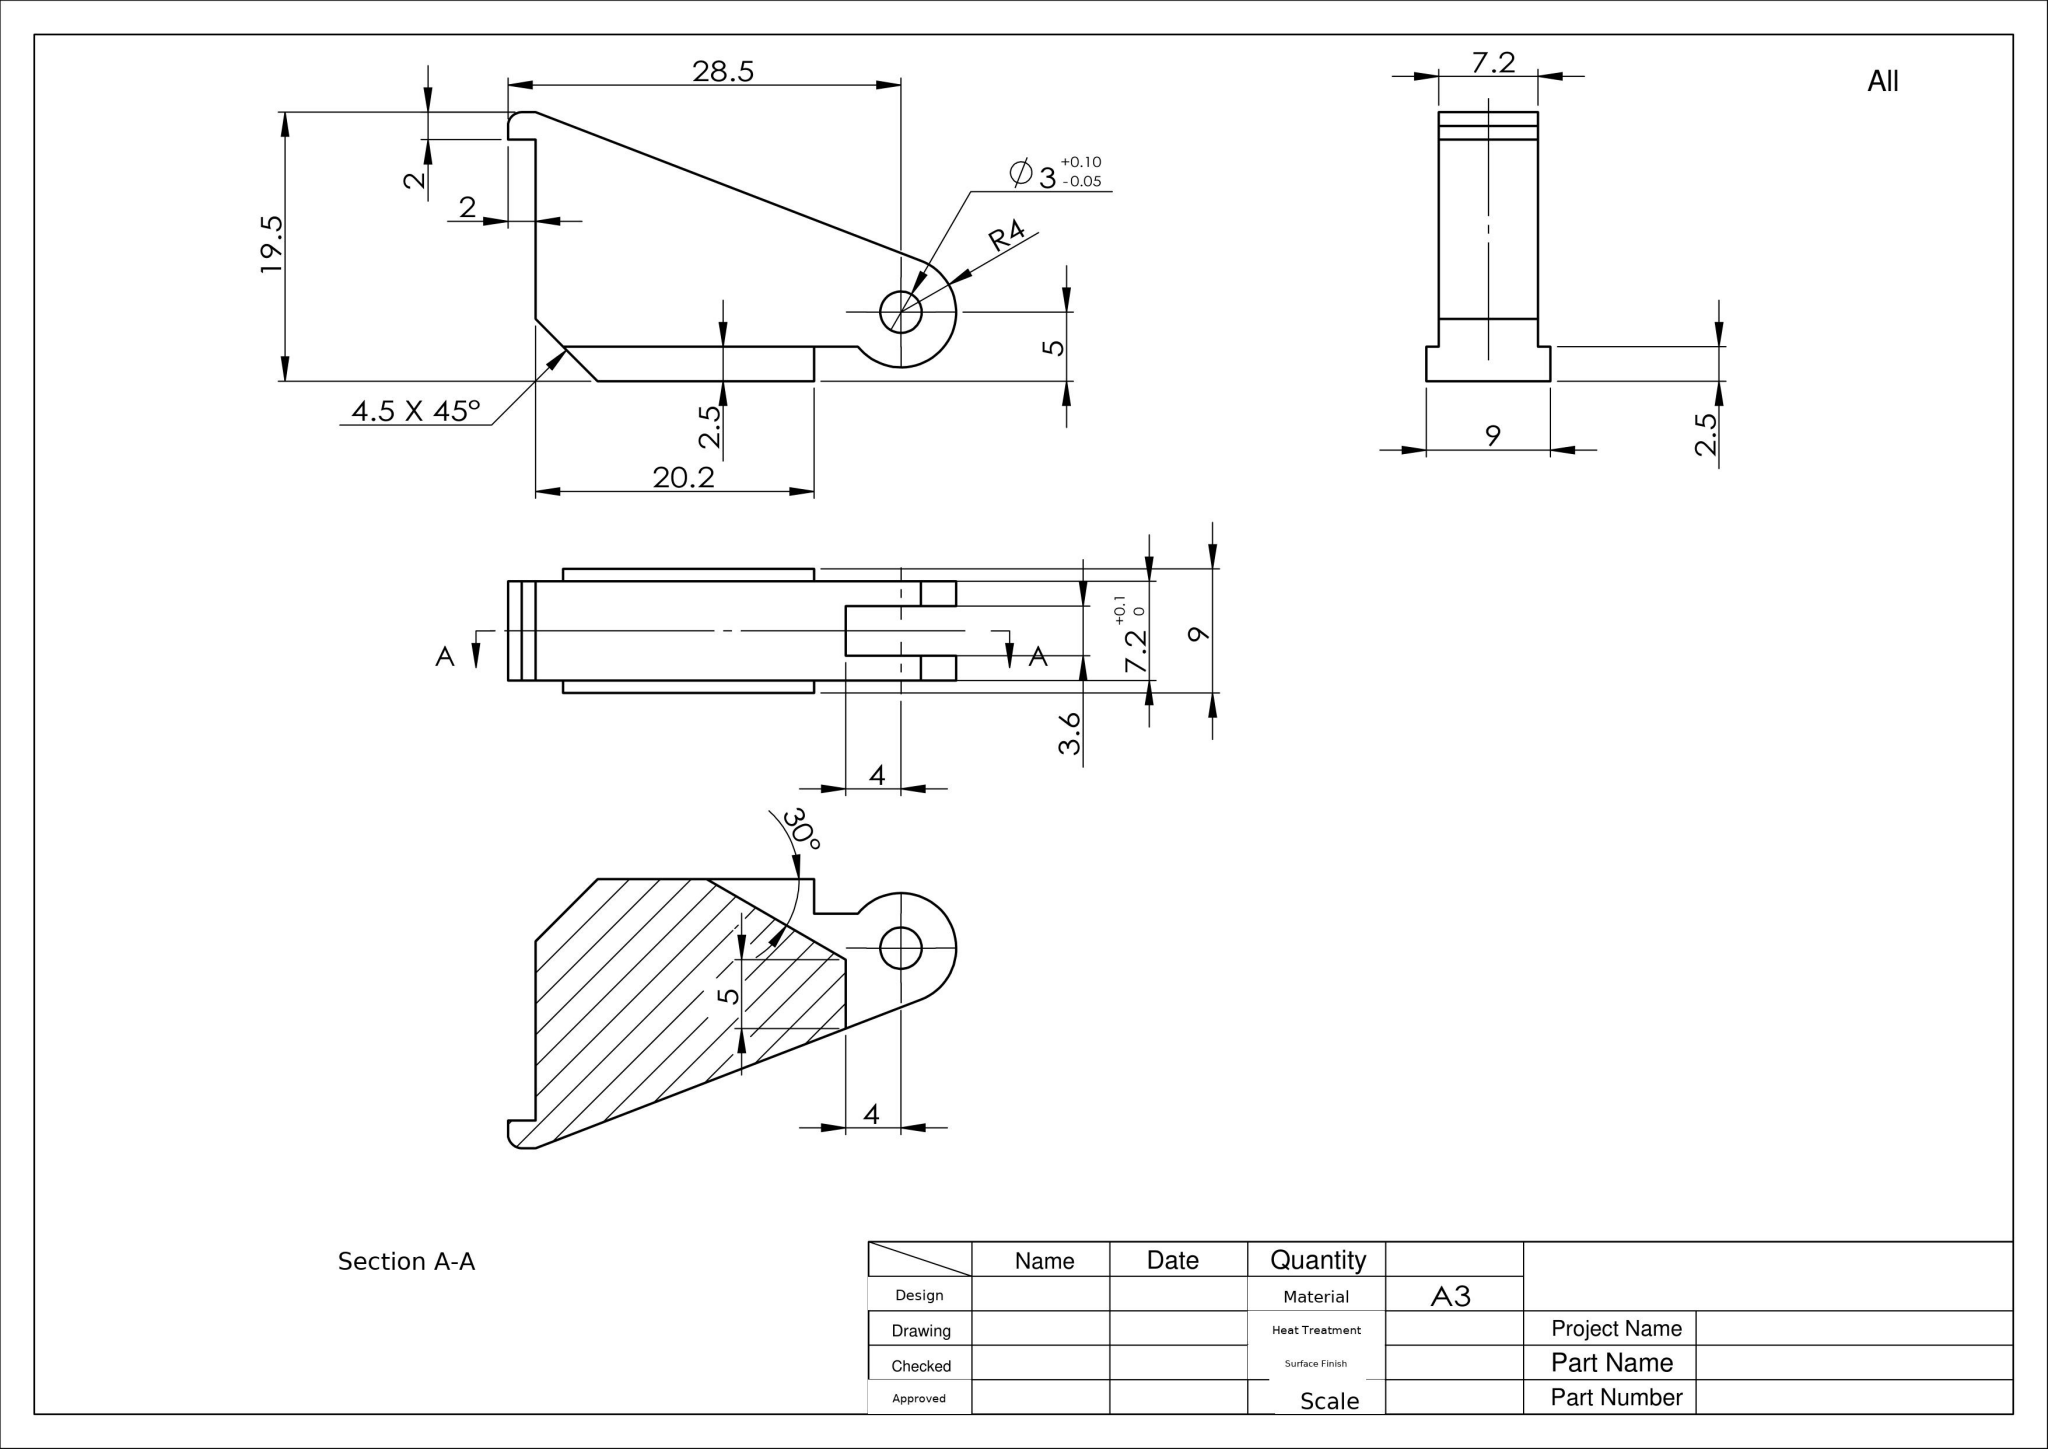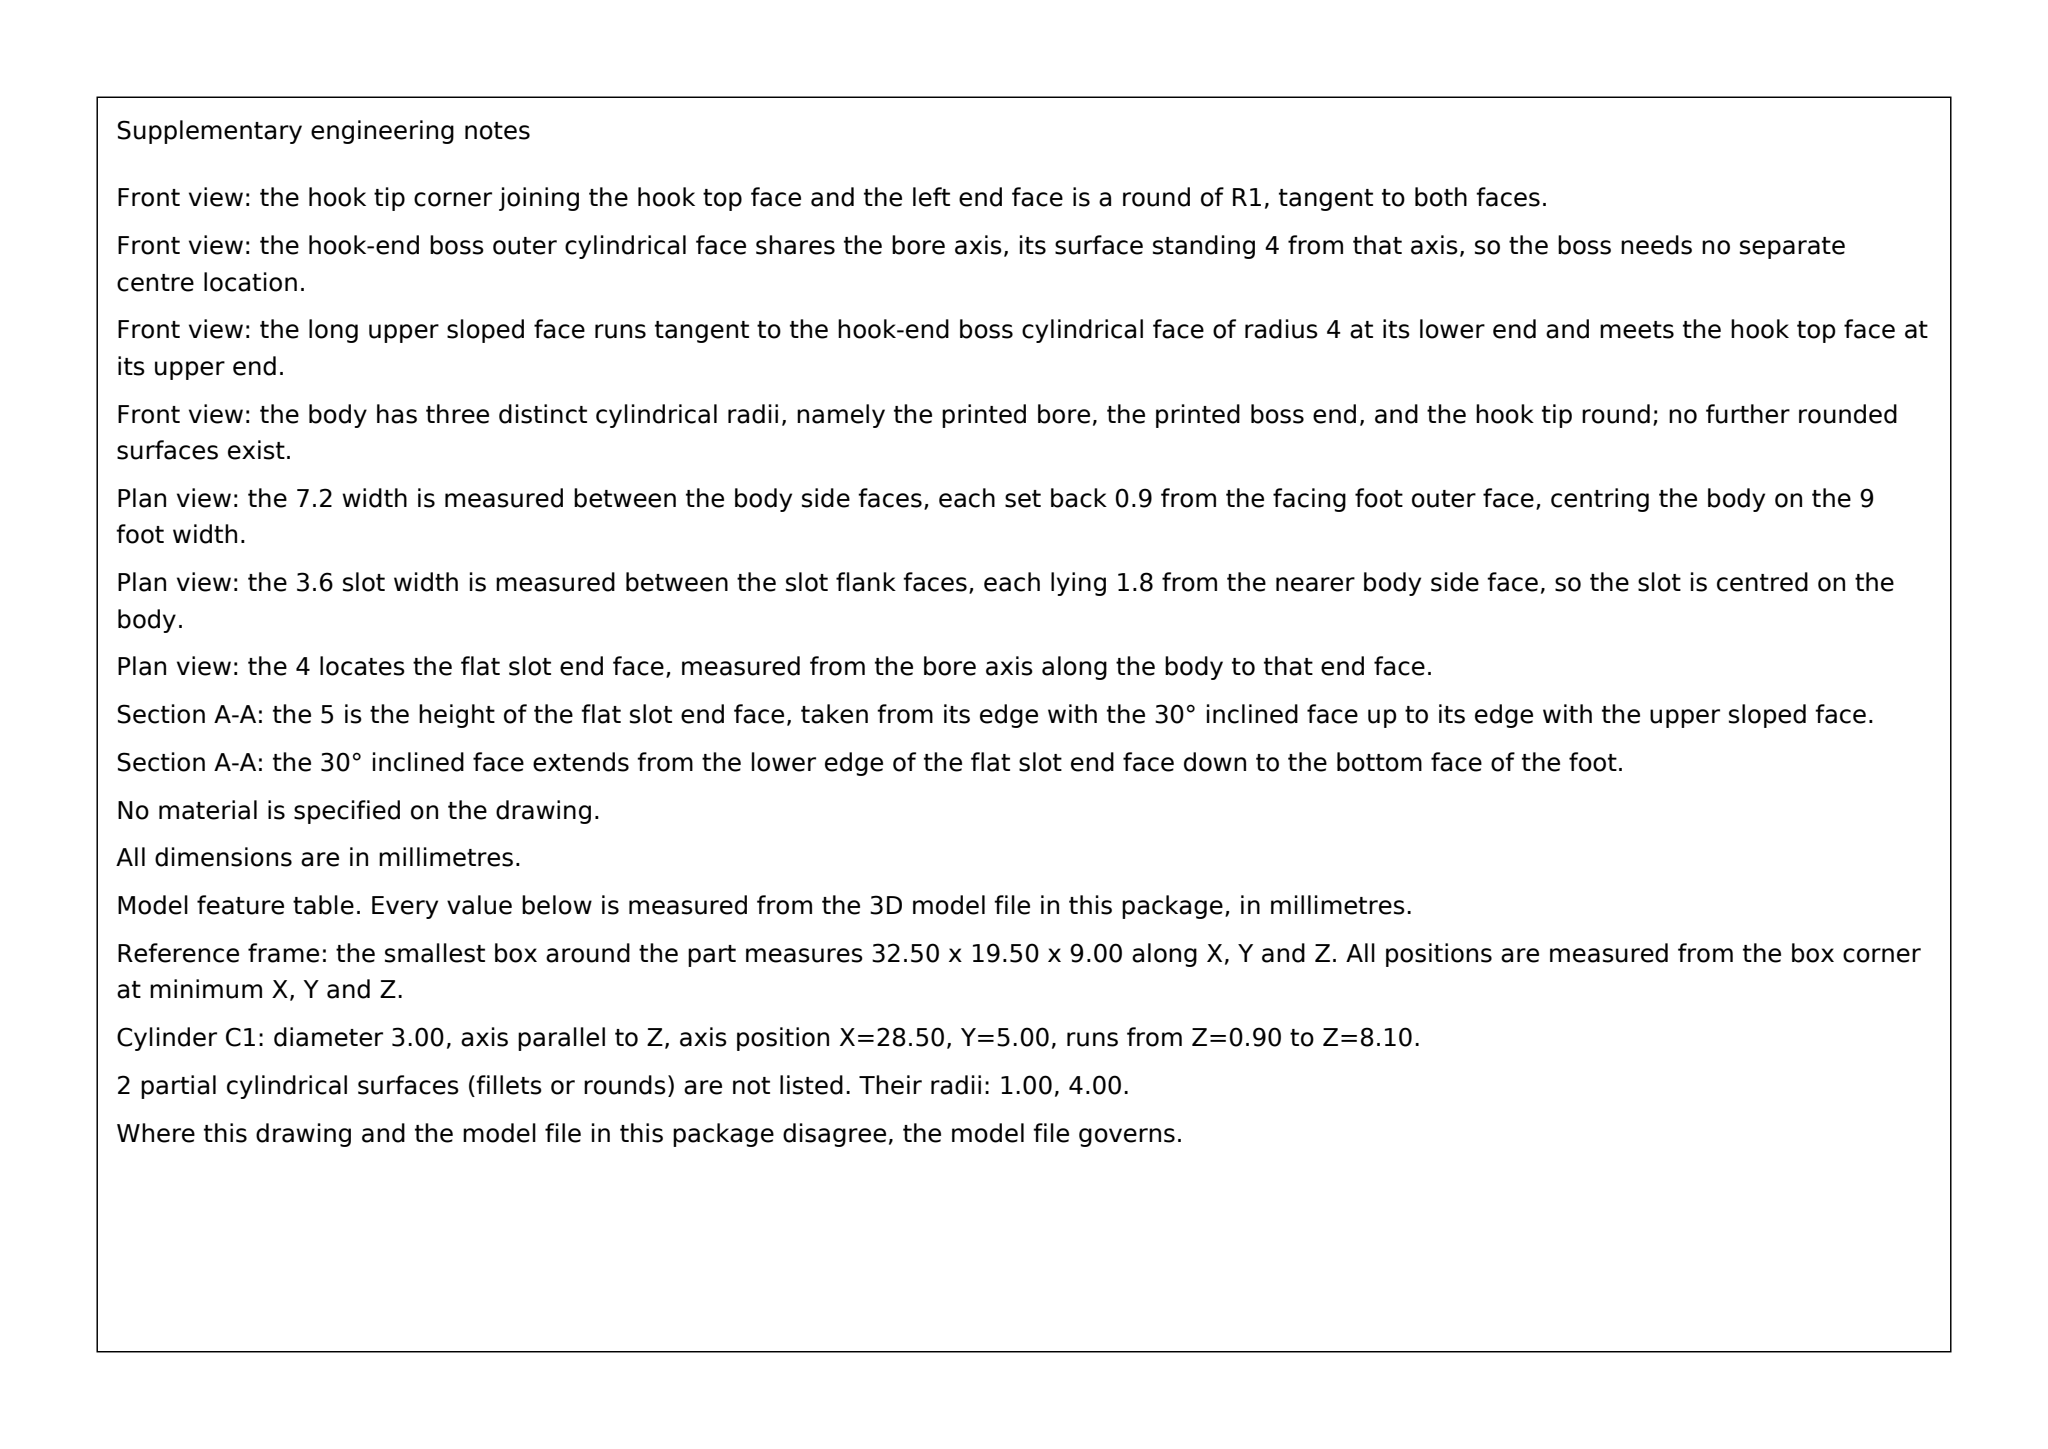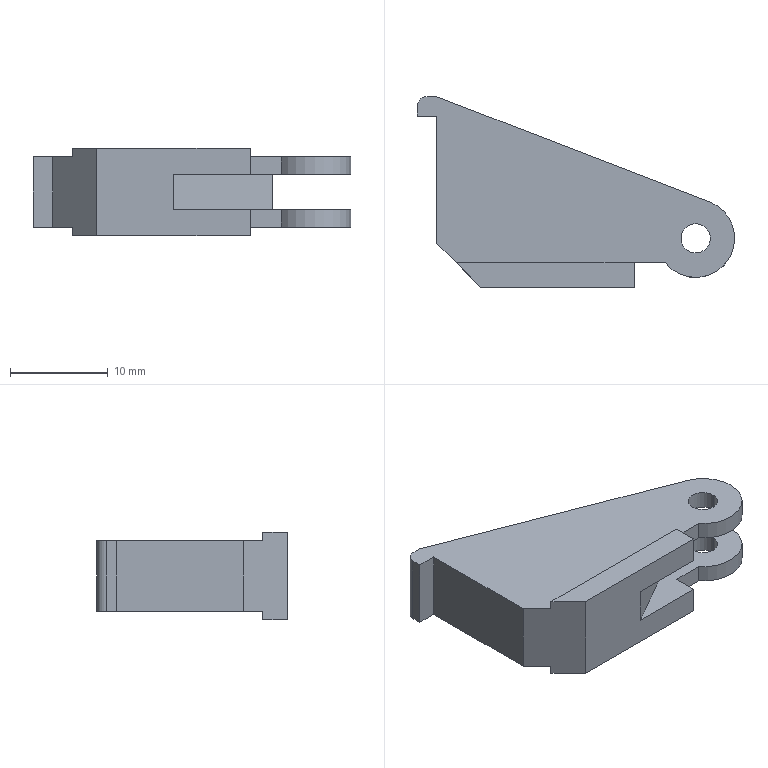Part | SolidWorks | mm | material A3 | 1 solid | 28 faces | box 32.5 x 19.5 x 9 mm | volume 2547 mm3 | plane 21 | cylinder 7 | commonest cylinder face diameters 3 x4 8 x2 2 x1
Drawing notes:
Ø2 hole, 7.2 deep, center located 1 from left end face and 1 from top face (18.5 from bottom face) | from the solid: cylinders[dia,axis,pos_other_axes,length]: [2.0,"z",[1.0,18.5],7.2] with bbox_xyz [32.5,19.5,9.0]
CORNER ROUND R1 (Ø2 FULL ROUND) AT TOP LEFT CORNER, CENTRE 1 FROM LEFT EDGE AND 1 FROM TOP EDGE (18.5 ABOVE BOTTOM), FULL 7.2 THICKNESS | from the solid: cylinders[dia 2.0, axis z, pos (1.0, 18.5), length 7.2, count 1]; axis_planes x=0.0, x=2.0, y=17.5, y=19.5
build123d program:
from build123d import *

# Parameters (mm, degrees)
SKETCH1_R          = 1.5
EXTRUDE1_DEPTH     = 9
SKETCH2_W          = 9.874
SKETCH2_H          = 3.6
CUT_EXTRUDE1_DEPTH = 36.686
CUT_EXTRUDE2_DEPTH = 1.8
CUT_EXTRUDE3_START = -0.9
CUT_EXTRUDE3_DEPTH = 0.9
CUT_EXTRUDE4_DEPTH = 0.9
FILLET1_R          = 1


with BuildPart() as part:
    # Sketch1 → Extrude1 (new body)
    with BuildSketch(Plane.XY):
        with BuildLine():
            Line((1.438, 3.732), (-26.5, 14.5))
            Line((-26.5, 14.5), (-28.5, 14.5))
            Line((-28.5, 14.5), (-28.5, 12.5))
            Line((-28.5, 12.5), (-26.5, 12.5))
            Line((-26.5, 12.5), (-26.5, -0.5))
            Line((-26.5, -0.5), (-22, -5))
            Line((-22, -5), (-6.3, -5))
            Line((-6.3, -5), (-6.3, -2.5))
            Line((-6.3, -2.5), (-3.122, -2.5))
            ThreePointArc((-3.122, -2.5), (3.228, -2.362), (1.438, 3.732))
        make_face()
        Circle(SKETCH1_R, mode=Mode.SUBTRACT)
    extrude(amount=EXTRUDE1_DEPTH)

    # Sketch2 → Cut-Extrude1 (cut, through all)
    with BuildSketch(Plane.XZ.offset(5)):
        with Locations((0.9369, 4.5)):
            Rectangle(SKETCH2_W, SKETCH2_H)
    extrude(amount=-CUT_EXTRUDE1_DEPTH, mode=Mode.SUBTRACT)

    # Sketch3 → Cut-Extrude2 (cut, symmetric)
    with BuildSketch(Plane(origin=(0, 0, 4.5), x_dir=(-1, 0, 0), z_dir=(0, 0, -1))):
        Polygon((4, -5), (4, 0.8284), (14.095, -5), align=None)
    extrude(amount=CUT_EXTRUDE2_DEPTH, both=True, mode=Mode.SUBTRACT)

    # Sketch4 → Cut-Extrude3 (cut)
    with BuildSketch(Plane.XY.offset(9).offset(CUT_EXTRUDE3_START)):
        with BuildLine():
            Line((-26.5, -0.5), (-24.5, -2.5))
            Line((-24.5, -2.5), (-3.122, -2.5))
            ThreePointArc((-3.122, -2.5), (3.228, -2.362), (1.438, 3.732))
            Line((1.438, 3.732), (-26.5, 14.5))
            Line((-26.5, 14.5), (-28.5, 14.5))
            Line((-28.5, 14.5), (-28.5, 12.5))
            Line((-28.5, 12.5), (-26.5, 12.5))
            Line((-26.5, 12.5), (-26.5, -0.5))
        make_face()
    extrude(amount=CUT_EXTRUDE3_DEPTH, mode=Mode.SUBTRACT)

    # Sketch5 → Cut-Extrude4 (cut)
    with BuildSketch(Plane(origin=(0, 0, 0), x_dir=(-1, 0, 0), z_dir=(0, 0, -1))):
        with BuildLine():
            Line((6.3, -2.5), (3.122, -2.5))
            ThreePointArc((3.122, -2.5), (-3.228, -2.362), (-1.438, 3.732))
            Line((-1.438, 3.732), (26.5, 14.5))
            Line((26.5, 14.5), (28.5, 14.5))
            Line((28.5, 14.5), (28.5, 12.5))
            Line((28.5, 12.5), (26.5, 12.5))
            Line((26.5, 12.5), (26.5, -0.5))
            Line((26.5, -0.5), (24.5, -2.5))
            Line((24.5, -2.5), (6.3, -2.5))
        make_face()
    extrude(amount=-CUT_EXTRUDE4_DEPTH, mode=Mode.SUBTRACT)

    # Fillet1
    fillet1_edges = [part.edges().sort_by_distance(p)[0] for p in [
        (-28.5, 14.5, 4.5),
    ]]
    fillet(fillet1_edges, radius=FILLET1_R)


solid = part.part